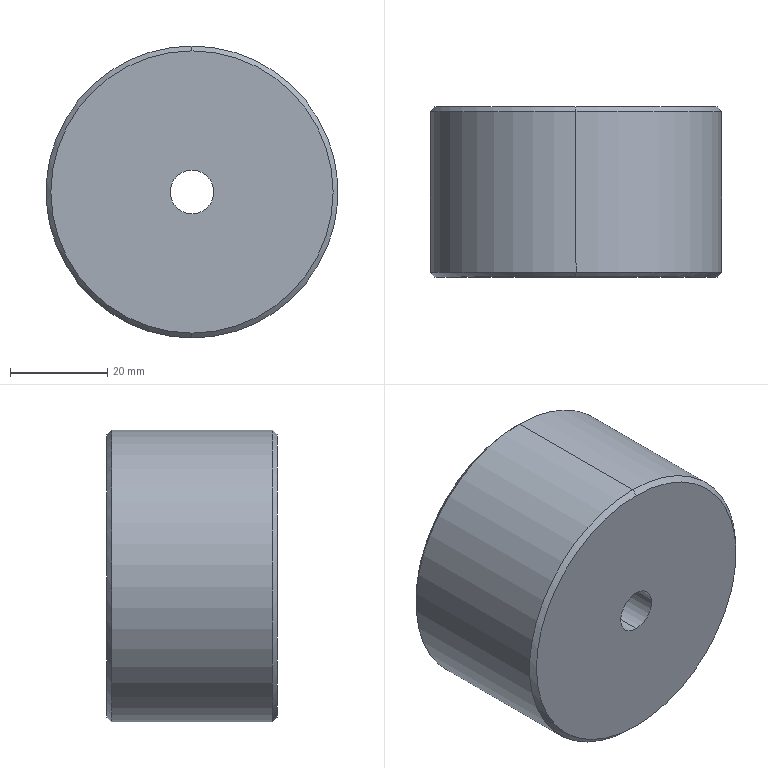Component | SolidWorks | MA060.03.03-10-3 | 1 solid | 15 faces | box 60 x 35 x 60 mm | volume 75578 mm3 | cone 6 | cylinder 6 | plane 3 | commonest cylinder face diameters 15 x2 9 x2 60 x2 | material Polyurethane
build123d program:
from build123d import *

# Parameters (mm, degrees)
SKETCH1_W                                            = 30
SKETCH1_H                                            = 35
HOLE_SIZE_ACCORDING_TO_TYPE_1_OF_HEX_SOC_D           = 9
HOLE_SIZE_ACCORDING_TO_TYPE_1_OF_HEX_SOC_CBORE_D     = 15
HOLE_SIZE_ACCORDING_TO_TYPE_1_OF_HEX_SOC_CBORE_DEPTH = 28
CHAMFER1_SIZE                                        = 20
CHAMFER2_SIZE                                        = 1


with BuildPart() as part:
    # Sketch1 → Revolve1 (revolve)
    with BuildSketch(Plane.XY, mode=Mode.PRIVATE) as revolve1_sk:
        with Locations((15, 17.5)):
            Rectangle(SKETCH1_W, SKETCH1_H)
    revolve(revolve1_sk.sketch.rotate(Axis((0, 0, 0), (0, 1, 0)), 90), axis=Axis((0, 0, 0), (0, 1, 0)))

    # Hole Size According to Type 1 of Hex Soc (through all)
    with Locations(Plane(origin=(0, 35, 0), x_dir=(-1, 0, 0), z_dir=(0, 1, 0))):
        with Locations((0, 0)):
            CounterBoreHole(HOLE_SIZE_ACCORDING_TO_TYPE_1_OF_HEX_SOC_D / 2, HOLE_SIZE_ACCORDING_TO_TYPE_1_OF_HEX_SOC_CBORE_D / 2, HOLE_SIZE_ACCORDING_TO_TYPE_1_OF_HEX_SOC_CBORE_DEPTH)

    # Chamfer1
    chamfer1_edges = [part.edges().sort_by_distance(p)[0] for p in [
        (7.5, 35, 0),
    ]]
    chamfer(chamfer1_edges, length=CHAMFER1_SIZE)

    # Chamfer2
    chamfer2_edges = [part.edges().sort_by_distance(p)[0] for p in [
        (0, 0, 30),
        (0, 35, 30),
    ]]
    chamfer(chamfer2_edges, length=CHAMFER2_SIZE)


solid = part.part

# Placed as in the assembly
solid = solid.moved(Location((263.711, 172.053, -96.036), (0, 0, 0)))
STEP:
#1=COLOUR_RGB('',0.7922,0.8196,0.9333);
#2=FILL_AREA_STYLE_COLOUR('',#1);
#3=FILL_AREA_STYLE('',(#2));
#4=SURFACE_STYLE_FILL_AREA(#3);
#5=SURFACE_SIDE_STYLE('',(#4));
#6=SURFACE_STYLE_USAGE(.BOTH.,#5);
#7=PRESENTATION_STYLE_ASSIGNMENT((#6));
#8=CARTESIAN_POINT('',(10.382,8.152,-4.923));
#9=VERTEX_POINT('',#8);
#10=CARTESIAN_POINT('',(10.382,8.152,-2.639));
#11=VERTEX_POINT('',#10);
#12=CARTESIAN_POINT('',(10.382,8.152,-3.781));
#13=DIRECTION('',(0.,1.,0.));
#14=DIRECTION('',(0.,0.,-1.));
#15=AXIS2_PLACEMENT_3D('',#12,#13,#14);
#16=CIRCLE('',#15,1.142);
#17=EDGE_CURVE('',#9,#11,#16,.T.);
#18=ORIENTED_EDGE('',*,*,#17,.F.);
#19=CARTESIAN_POINT('',(10.382,8.112,-4.962));
#20=VERTEX_POINT('',#19);
#21=CARTESIAN_POINT('',(10.382,8.112,-4.962));
#22=DIRECTION('',(-0.,-0.7071,-0.7071));
#23=VECTOR('',#22,39.37);
#24=LINE('',#21,#23);
#25=EDGE_CURVE('',#9,#20,#24,.T.);
#26=ORIENTED_EDGE('',*,*,#25,.T.);
#27=CARTESIAN_POINT('',(10.382,8.112,-2.6));
#28=VERTEX_POINT('',#27);
#29=CARTESIAN_POINT('',(10.382,8.112,-3.781));
#30=DIRECTION('',(-0.,-1.,-0.));
#31=DIRECTION('',(0.,0.,-1.));
#32=AXIS2_PLACEMENT_3D('',#29,#30,#31);
#33=CIRCLE('',#32,1.181);
#34=EDGE_CURVE('',#28,#20,#33,.T.);
#35=ORIENTED_EDGE('',*,*,#34,.F.);
#36=CARTESIAN_POINT('',(10.382,8.112,-2.6));
#37=DIRECTION('',(-0.,-0.7071,0.7071));
#38=VECTOR('',#37,39.37);
#39=LINE('',#36,#38);
#40=EDGE_CURVE('',#11,#28,#39,.T.);
#41=ORIENTED_EDGE('',*,*,#40,.F.);
#42=EDGE_LOOP('',(#18,#26,#35,#41));
#43=FACE_OUTER_BOUND('',#42,.T.);
#44=CARTESIAN_POINT('',(10.382,8.112,-3.781));
#45=DIRECTION('',(-0.,-1.,-0.));
#46=DIRECTION('',(0.,0.,1.));
#47=AXIS2_PLACEMENT_3D('',#44,#45,#46);
#48=CONICAL_SURFACE('',#47,1.181,0.7854);
#49=ADVANCED_FACE('',(#43),#48,.T.);
#50=CARTESIAN_POINT('',(10.382,6.774,-2.639));
#51=VERTEX_POINT('',#50);
#52=CARTESIAN_POINT('',(10.382,6.774,-4.923));
#53=VERTEX_POINT('',#52);
#54=CARTESIAN_POINT('',(10.382,6.774,-3.781));
#55=DIRECTION('',(-0.,-1.,-0.));
#56=DIRECTION('',(0.,0.,1.));
#57=AXIS2_PLACEMENT_3D('',#54,#55,#56);
#58=CIRCLE('',#57,1.142);
#59=EDGE_CURVE('',#51,#53,#58,.T.);
#60=ORIENTED_EDGE('',*,*,#59,.F.);
#61=CARTESIAN_POINT('',(10.382,6.813,-2.6));
#62=VERTEX_POINT('',#61);
#63=CARTESIAN_POINT('',(10.382,6.774,-2.639));
#64=DIRECTION('',(-0.,0.7071,0.7071));
#65=VECTOR('',#64,39.37);
#66=LINE('',#63,#65);
#67=EDGE_CURVE('',#51,#62,#66,.T.);
#68=ORIENTED_EDGE('',*,*,#67,.T.);
#69=CARTESIAN_POINT('',(10.382,6.813,-4.962));
#70=VERTEX_POINT('',#69);
#71=CARTESIAN_POINT('',(10.382,6.813,-3.781));
#72=DIRECTION('',(0.,1.,0.));
#73=DIRECTION('',(0.,0.,1.));
#74=AXIS2_PLACEMENT_3D('',#71,#72,#73);
#75=CIRCLE('',#74,1.181);
#76=EDGE_CURVE('',#70,#62,#75,.T.);
#77=ORIENTED_EDGE('',*,*,#76,.F.);
#78=CARTESIAN_POINT('',(10.382,6.774,-4.923));
#79=DIRECTION('',(0.,0.7071,-0.7071));
#80=VECTOR('',#79,39.37);
#81=LINE('',#78,#80);
#82=EDGE_CURVE('',#53,#70,#81,.T.);
#83=ORIENTED_EDGE('',*,*,#82,.F.);
#84=EDGE_LOOP('',(#60,#68,#77,#83));
#85=FACE_OUTER_BOUND('',#84,.T.);
#86=CARTESIAN_POINT('',(10.382,6.774,-3.781));
#87=DIRECTION('',(0.,1.,0.));
#88=DIRECTION('',(0.,0.,-1.));
#89=AXIS2_PLACEMENT_3D('',#86,#87,#88);
#90=CONICAL_SURFACE('',#89,1.142,0.7854);
#91=ADVANCED_FACE('',(#85),#90,.T.);
#92=CARTESIAN_POINT('',(10.382,7.364,-3.486));
#93=VERTEX_POINT('',#92);
#94=CARTESIAN_POINT('',(10.382,7.364,-4.076));
#95=VERTEX_POINT('',#94);
#96=CARTESIAN_POINT('',(10.382,7.364,-3.781));
#97=DIRECTION('',(0.,1.,0.));
#98=DIRECTION('',(0.,0.,-1.));
#99=AXIS2_PLACEMENT_3D('',#96,#97,#98);
#100=CIRCLE('',#99,0.2953);
#101=EDGE_CURVE('',#93,#95,#100,.T.);
#102=ORIENTED_EDGE('',*,*,#101,.F.);
#103=CARTESIAN_POINT('',(10.382,8.152,-2.698));
#104=VERTEX_POINT('',#103);
#105=CARTESIAN_POINT('',(10.382,7.364,-3.486));
#106=DIRECTION('',(-0.,0.7071,0.7071));
#107=VECTOR('',#106,39.37);
#108=LINE('',#105,#107);
#109=EDGE_CURVE('',#93,#104,#108,.T.);
#110=ORIENTED_EDGE('',*,*,#109,.T.);
#111=CARTESIAN_POINT('',(10.382,8.152,-4.864));
#112=VERTEX_POINT('',#111);
#113=CARTESIAN_POINT('',(10.382,8.152,-3.781));
#114=DIRECTION('',(-0.,-1.,-0.));
#115=DIRECTION('',(0.,0.,-1.));
#116=AXIS2_PLACEMENT_3D('',#113,#114,#115);
#117=CIRCLE('',#116,1.083);
#118=EDGE_CURVE('',#112,#104,#117,.T.);
#119=ORIENTED_EDGE('',*,*,#118,.F.);
#120=CARTESIAN_POINT('',(10.382,7.364,-4.076));
#121=DIRECTION('',(0.,0.7071,-0.7071));
#122=VECTOR('',#121,39.37);
#123=LINE('',#120,#122);
#124=EDGE_CURVE('',#95,#112,#123,.T.);
#125=ORIENTED_EDGE('',*,*,#124,.F.);
#126=EDGE_LOOP('',(#102,#110,#119,#125));
#127=FACE_OUTER_BOUND('',#126,.T.);
#128=CARTESIAN_POINT('',(10.382,7.364,-3.781));
#129=DIRECTION('',(0.,1.,0.));
#130=DIRECTION('',(0.,0.,-1.));
#131=AXIS2_PLACEMENT_3D('',#128,#129,#130);
#132=CONICAL_SURFACE('',#131,0.2953,0.7854);
#133=ADVANCED_FACE('',(#127),#132,.F.);
#134=CARTESIAN_POINT('',(10.382,7.049,-3.486));
#135=VERTEX_POINT('',#134);
#136=CARTESIAN_POINT('',(10.382,7.049,-4.076));
#137=VERTEX_POINT('',#136);
#138=CARTESIAN_POINT('',(10.382,7.049,-3.781));
#139=DIRECTION('',(0.,1.,0.));
#140=DIRECTION('',(0.,0.,-1.));
#141=AXIS2_PLACEMENT_3D('',#138,#139,#140);
#142=CIRCLE('',#141,0.2953);
#143=EDGE_CURVE('',#135,#137,#142,.T.);
#144=ORIENTED_EDGE('',*,*,#143,.F.);
#145=CARTESIAN_POINT('',(10.382,8.152,-3.486));
#146=DIRECTION('',(0.,1.,0.));
#147=VECTOR('',#146,39.37);
#148=LINE('',#145,#147);
#149=EDGE_CURVE('',#135,#93,#148,.T.);
#150=ORIENTED_EDGE('',*,*,#149,.T.);
#151=ORIENTED_EDGE('',*,*,#101,.T.);
#152=CARTESIAN_POINT('',(10.382,8.152,-4.076));
#153=DIRECTION('',(0.,1.,0.));
#154=VECTOR('',#153,39.37);
#155=LINE('',#152,#154);
#156=EDGE_CURVE('',#137,#95,#155,.T.);
#157=ORIENTED_EDGE('',*,*,#156,.F.);
#158=EDGE_LOOP('',(#144,#150,#151,#157));
#159=FACE_OUTER_BOUND('',#158,.T.);
#160=CARTESIAN_POINT('',(10.382,8.152,-3.781));
#161=DIRECTION('',(0.,1.,0.));
#162=DIRECTION('',(0.,0.,-1.));
#163=AXIS2_PLACEMENT_3D('',#160,#161,#162);
#164=CYLINDRICAL_SURFACE('',#163,0.2953);
#165=ADVANCED_FACE('',(#159),#164,.F.);
#166=CARTESIAN_POINT('',(10.382,6.774,-3.604));
#167=VERTEX_POINT('',#166);
#168=CARTESIAN_POINT('',(10.382,6.774,-3.958));
#169=VERTEX_POINT('',#168);
#170=CARTESIAN_POINT('',(10.382,6.774,-3.781));
#171=DIRECTION('',(0.,1.,0.));
#172=DIRECTION('',(0.,0.,-1.));
#173=AXIS2_PLACEMENT_3D('',#170,#171,#172);
#174=CIRCLE('',#173,0.1772);
#175=EDGE_CURVE('',#167,#169,#174,.T.);
#176=ORIENTED_EDGE('',*,*,#175,.F.);
#177=CARTESIAN_POINT('',(10.382,7.049,-3.604));
#178=VERTEX_POINT('',#177);
#179=CARTESIAN_POINT('',(10.382,8.152,-3.604));
#180=DIRECTION('',(0.,1.,0.));
#181=VECTOR('',#180,39.37);
#182=LINE('',#179,#181);
#183=EDGE_CURVE('',#167,#178,#182,.T.);
#184=ORIENTED_EDGE('',*,*,#183,.T.);
#185=CARTESIAN_POINT('',(10.382,7.049,-3.958));
#186=VERTEX_POINT('',#185);
#187=CARTESIAN_POINT('',(10.382,7.049,-3.781));
#188=DIRECTION('',(0.,1.,0.));
#189=DIRECTION('',(0.,0.,-1.));
#190=AXIS2_PLACEMENT_3D('',#187,#188,#189);
#191=CIRCLE('',#190,0.1772);
#192=EDGE_CURVE('',#178,#186,#191,.T.);
#193=ORIENTED_EDGE('',*,*,#192,.T.);
#194=CARTESIAN_POINT('',(10.382,8.152,-3.958));
#195=DIRECTION('',(0.,1.,0.));
#196=VECTOR('',#195,39.37);
#197=LINE('',#194,#196);
#198=EDGE_CURVE('',#169,#186,#197,.T.);
#199=ORIENTED_EDGE('',*,*,#198,.F.);
#200=EDGE_LOOP('',(#176,#184,#193,#199));
#201=FACE_OUTER_BOUND('',#200,.T.);
#202=CARTESIAN_POINT('',(10.382,8.152,-3.781));
#203=DIRECTION('',(0.,1.,0.));
#204=DIRECTION('',(0.,0.,-1.));
#205=AXIS2_PLACEMENT_3D('',#202,#203,#204);
#206=CYLINDRICAL_SURFACE('',#205,0.1772);
#207=ADVANCED_FACE('',(#201),#206,.F.);
#208=ORIENTED_EDGE('',*,*,#34,.T.);
#209=CARTESIAN_POINT('',(10.382,6.774,-4.962));
#210=DIRECTION('',(-0.,-1.,-0.));
#211=VECTOR('',#210,39.37);
#212=LINE('',#209,#211);
#213=EDGE_CURVE('',#20,#70,#212,.T.);
#214=ORIENTED_EDGE('',*,*,#213,.T.);
#215=ORIENTED_EDGE('',*,*,#76,.T.);
#216=CARTESIAN_POINT('',(10.382,6.774,-2.6));
#217=DIRECTION('',(-0.,-1.,-0.));
#218=VECTOR('',#217,39.37);
#219=LINE('',#216,#218);
#220=EDGE_CURVE('',#28,#62,#219,.T.);
#221=ORIENTED_EDGE('',*,*,#220,.F.);
#222=EDGE_LOOP('',(#208,#214,#215,#221));
#223=FACE_OUTER_BOUND('',#222,.T.);
#224=CARTESIAN_POINT('',(10.382,6.774,-3.781));
#225=DIRECTION('',(-0.,-1.,-0.));
#226=DIRECTION('',(0.,0.,1.));
#227=AXIS2_PLACEMENT_3D('',#224,#225,#226);
#228=CYLINDRICAL_SURFACE('',#227,1.181);
#229=ADVANCED_FACE('',(#223),#228,.T.);
#230=CARTESIAN_POINT('',(10.382,8.152,-3.781));
#231=DIRECTION('',(0.,1.,0.));
#232=DIRECTION('',(0.,0.,-1.));
#233=AXIS2_PLACEMENT_3D('',#230,#231,#232);
#234=CIRCLE('',#233,1.142);
#235=EDGE_CURVE('',#11,#9,#234,.T.);
#236=ORIENTED_EDGE('',*,*,#235,.T.);
#237=ORIENTED_EDGE('',*,*,#17,.T.);
#238=EDGE_LOOP('',(#236,#237));
#239=FACE_OUTER_BOUND('',#238,.T.);
#240=ORIENTED_EDGE('',*,*,#118,.T.);
#241=CARTESIAN_POINT('',(10.382,8.152,-3.781));
#242=DIRECTION('',(-0.,-1.,-0.));
#243=DIRECTION('',(-0.,0.,-1.));
#244=AXIS2_PLACEMENT_3D('',#241,#242,#243);
#245=CIRCLE('',#244,1.083);
#246=EDGE_CURVE('',#104,#112,#245,.T.);
#247=ORIENTED_EDGE('',*,*,#246,.T.);
#248=EDGE_LOOP('',(#240,#247));
#249=FACE_BOUND('',#248,.T.);
#250=CARTESIAN_POINT('',(10.382,8.152,-3.781));
#251=DIRECTION('',(0.,1.,-0.));
#252=DIRECTION('',(0.,-0.,-1.));
#253=AXIS2_PLACEMENT_3D('',#250,#251,#252);
#254=PLANE('',#253);
#255=ADVANCED_FACE('',(#239,#249),#254,.T.);
#256=ORIENTED_EDGE('',*,*,#213,.F.);
#257=CARTESIAN_POINT('',(10.382,8.112,-3.781));
#258=DIRECTION('',(-0.,-1.,-0.));
#259=DIRECTION('',(0.,0.,-1.));
#260=AXIS2_PLACEMENT_3D('',#257,#258,#259);
#261=CIRCLE('',#260,1.181);
#262=EDGE_CURVE('',#20,#28,#261,.T.);
#263=ORIENTED_EDGE('',*,*,#262,.T.);
#264=ORIENTED_EDGE('',*,*,#220,.T.);
#265=CARTESIAN_POINT('',(10.382,6.813,-3.781));
#266=DIRECTION('',(0.,1.,0.));
#267=DIRECTION('',(0.,0.,1.));
#268=AXIS2_PLACEMENT_3D('',#265,#266,#267);
#269=CIRCLE('',#268,1.181);
#270=EDGE_CURVE('',#62,#70,#269,.T.);
#271=ORIENTED_EDGE('',*,*,#270,.T.);
#272=EDGE_LOOP('',(#256,#263,#264,#271));
#273=FACE_OUTER_BOUND('',#272,.T.);
#274=CARTESIAN_POINT('',(10.382,6.774,-3.781));
#275=DIRECTION('',(-0.,-1.,-0.));
#276=DIRECTION('',(0.,0.,1.));
#277=AXIS2_PLACEMENT_3D('',#274,#275,#276);
#278=CYLINDRICAL_SURFACE('',#277,1.181);
#279=ADVANCED_FACE('',(#273),#278,.T.);
#280=CARTESIAN_POINT('',(10.382,6.774,-3.781));
#281=DIRECTION('',(-0.,-1.,-0.));
#282=DIRECTION('',(0.,0.,1.));
#283=AXIS2_PLACEMENT_3D('',#280,#281,#282);
#284=CIRCLE('',#283,1.142);
#285=EDGE_CURVE('',#53,#51,#284,.T.);
#286=ORIENTED_EDGE('',*,*,#285,.T.);
#287=ORIENTED_EDGE('',*,*,#59,.T.);
#288=EDGE_LOOP('',(#286,#287));
#289=FACE_OUTER_BOUND('',#288,.T.);
#290=CARTESIAN_POINT('',(10.382,6.774,-3.781));
#291=DIRECTION('',(0.,1.,0.));
#292=DIRECTION('',(0.,0.,-1.));
#293=AXIS2_PLACEMENT_3D('',#290,#291,#292);
#294=CIRCLE('',#293,0.1772);
#295=EDGE_CURVE('',#169,#167,#294,.T.);
#296=ORIENTED_EDGE('',*,*,#295,.T.);
#297=ORIENTED_EDGE('',*,*,#175,.T.);
#298=EDGE_LOOP('',(#296,#297));
#299=FACE_BOUND('',#298,.T.);
#300=CARTESIAN_POINT('',(10.382,6.774,-3.781));
#301=DIRECTION('',(-0.,-1.,0.));
#302=DIRECTION('',(0.,0.,1.));
#303=AXIS2_PLACEMENT_3D('',#300,#301,#302);
#304=PLANE('',#303);
#305=ADVANCED_FACE('',(#289,#299),#304,.T.);
#306=ORIENTED_EDGE('',*,*,#183,.F.);
#307=ORIENTED_EDGE('',*,*,#295,.F.);
#308=ORIENTED_EDGE('',*,*,#198,.T.);
#309=CARTESIAN_POINT('',(10.382,7.049,-3.781));
#310=DIRECTION('',(0.,1.,0.));
#311=DIRECTION('',(0.,0.,-1.));
#312=AXIS2_PLACEMENT_3D('',#309,#310,#311);
#313=CIRCLE('',#312,0.1772);
#314=EDGE_CURVE('',#186,#178,#313,.T.);
#315=ORIENTED_EDGE('',*,*,#314,.T.);
#316=EDGE_LOOP('',(#306,#307,#308,#315));
#317=FACE_OUTER_BOUND('',#316,.T.);
#318=CARTESIAN_POINT('',(10.382,8.152,-3.781));
#319=DIRECTION('',(0.,1.,0.));
#320=DIRECTION('',(0.,0.,-1.));
#321=AXIS2_PLACEMENT_3D('',#318,#319,#320);
#322=CYLINDRICAL_SURFACE('',#321,0.1772);
#323=ADVANCED_FACE('',(#317),#322,.F.);
#324=ORIENTED_EDGE('',*,*,#314,.F.);
#325=ORIENTED_EDGE('',*,*,#192,.F.);
#326=EDGE_LOOP('',(#324,#325));
#327=FACE_BOUND('',#326,.T.);
#328=CARTESIAN_POINT('',(10.382,7.049,-3.781));
#329=DIRECTION('',(0.,1.,0.));
#330=DIRECTION('',(0.,0.,-1.));
#331=AXIS2_PLACEMENT_3D('',#328,#329,#330);
#332=CIRCLE('',#331,0.2953);
#333=EDGE_CURVE('',#137,#135,#332,.T.);
#334=ORIENTED_EDGE('',*,*,#333,.T.);
#335=ORIENTED_EDGE('',*,*,#143,.T.);
#336=EDGE_LOOP('',(#334,#335));
#337=FACE_OUTER_BOUND('',#336,.T.);
#338=CARTESIAN_POINT('',(10.205,7.049,-3.781));
#339=DIRECTION('',(-0.,-1.,0.));
#340=DIRECTION('',(0.,0.,1.));
#341=AXIS2_PLACEMENT_3D('',#338,#339,#340);
#342=PLANE('',#341);
#343=ADVANCED_FACE('',(#327,#337),#342,.F.);
#344=ORIENTED_EDGE('',*,*,#149,.F.);
#345=ORIENTED_EDGE('',*,*,#333,.F.);
#346=ORIENTED_EDGE('',*,*,#156,.T.);
#347=CARTESIAN_POINT('',(10.382,7.364,-3.781));
#348=DIRECTION('',(0.,1.,0.));
#349=DIRECTION('',(0.,0.,-1.));
#350=AXIS2_PLACEMENT_3D('',#347,#348,#349);
#351=CIRCLE('',#350,0.2953);
#352=EDGE_CURVE('',#95,#93,#351,.T.);
#353=ORIENTED_EDGE('',*,*,#352,.T.);
#354=EDGE_LOOP('',(#344,#345,#346,#353));
#355=FACE_OUTER_BOUND('',#354,.T.);
#356=CARTESIAN_POINT('',(10.382,8.152,-3.781));
#357=DIRECTION('',(0.,1.,0.));
#358=DIRECTION('',(0.,0.,-1.));
#359=AXIS2_PLACEMENT_3D('',#356,#357,#358);
#360=CYLINDRICAL_SURFACE('',#359,0.2953);
#361=ADVANCED_FACE('',(#355),#360,.F.);
#362=ORIENTED_EDGE('',*,*,#109,.F.);
#363=ORIENTED_EDGE('',*,*,#352,.F.);
#364=ORIENTED_EDGE('',*,*,#124,.T.);
#365=ORIENTED_EDGE('',*,*,#246,.F.);
#366=EDGE_LOOP('',(#362,#363,#364,#365));
#367=FACE_OUTER_BOUND('',#366,.T.);
#368=CARTESIAN_POINT('',(10.382,7.364,-3.781));
#369=DIRECTION('',(0.,1.,0.));
#370=DIRECTION('',(0.,0.,-1.));
#371=AXIS2_PLACEMENT_3D('',#368,#369,#370);
#372=CONICAL_SURFACE('',#371,0.2953,0.7854);
#373=ADVANCED_FACE('',(#367),#372,.F.);
#374=ORIENTED_EDGE('',*,*,#67,.F.);
#375=ORIENTED_EDGE('',*,*,#285,.F.);
#376=ORIENTED_EDGE('',*,*,#82,.T.);
#377=ORIENTED_EDGE('',*,*,#270,.F.);
#378=EDGE_LOOP('',(#374,#375,#376,#377));
#379=FACE_OUTER_BOUND('',#378,.T.);
#380=CARTESIAN_POINT('',(10.382,6.774,-3.781));
#381=DIRECTION('',(0.,1.,0.));
#382=DIRECTION('',(0.,0.,-1.));
#383=AXIS2_PLACEMENT_3D('',#380,#381,#382);
#384=CONICAL_SURFACE('',#383,1.142,0.7854);
#385=ADVANCED_FACE('',(#379),#384,.T.);
#386=ORIENTED_EDGE('',*,*,#25,.F.);
#387=ORIENTED_EDGE('',*,*,#235,.F.);
#388=ORIENTED_EDGE('',*,*,#40,.T.);
#389=ORIENTED_EDGE('',*,*,#262,.F.);
#390=EDGE_LOOP('',(#386,#387,#388,#389));
#391=FACE_OUTER_BOUND('',#390,.T.);
#392=CARTESIAN_POINT('',(10.382,8.112,-3.781));
#393=DIRECTION('',(-0.,-1.,-0.));
#394=DIRECTION('',(0.,0.,1.));
#395=AXIS2_PLACEMENT_3D('',#392,#393,#394);
#396=CONICAL_SURFACE('',#395,1.181,0.7854);
#397=ADVANCED_FACE('',(#391),#396,.T.);
#398=CLOSED_SHELL('',(#49,#91,#133,#165,#207,#229,#255,#279,#305,#323,#343,#361,#373,#385,#397));
#399=MANIFOLD_SOLID_BREP('',#398);
#400=STYLED_ITEM('',(#7),#399);
#401=(LENGTH_UNIT()NAMED_UNIT(*)SI_UNIT($,.METRE.));
#402=LENGTH_MEASURE_WITH_UNIT(LENGTH_MEASURE(0.0254),#401);
#403=DIMENSIONAL_EXPONENTS(1.,0.,0.,0.,0.,0.,0.);
#404=(CONVERSION_BASED_UNIT('',#402)LENGTH_UNIT()NAMED_UNIT(#403));
#405=UNCERTAINTY_MEASURE_WITH_UNIT(LENGTH_MEASURE(0.00001),#404,'','');
#406=(NAMED_UNIT(*)PLANE_ANGLE_UNIT()SI_UNIT($,.RADIAN.));
#407=(NAMED_UNIT(*)SI_UNIT($,.STERADIAN.)SOLID_ANGLE_UNIT());
#408=(GEOMETRIC_REPRESENTATION_CONTEXT(3)GLOBAL_UNCERTAINTY_ASSIGNED_CONTEXT((#405))GLOBAL_UNIT_ASSIGNED_CONTEXT((#404,#406,#407))REPRESENTATION_CONTEXT('',''));
#409=MECHANICAL_DESIGN_GEOMETRIC_PRESENTATION_REPRESENTATION('',(#400),#408);
#410=PRESENTATION_LAYER_ASSIGNMENT('','',(#400));
#411=CARTESIAN_POINT('',(0.,0.,0.));
#412=DIRECTION('',(0.,0.,1.));
#413=DIRECTION('',(1.,0.,0.));
#414=AXIS2_PLACEMENT_3D('',#411,#412,#413);
#415=(LENGTH_UNIT()NAMED_UNIT(*)SI_UNIT($,.METRE.));
#416=LENGTH_MEASURE_WITH_UNIT(LENGTH_MEASURE(0.0254),#415);
#417=DIMENSIONAL_EXPONENTS(1.,0.,0.,0.,0.,0.,0.);
#418=(CONVERSION_BASED_UNIT('',#416)LENGTH_UNIT()NAMED_UNIT(#417));
#419=UNCERTAINTY_MEASURE_WITH_UNIT(LENGTH_MEASURE(0.00001),#418,'','');
#420=(NAMED_UNIT(*)PLANE_ANGLE_UNIT()SI_UNIT($,.RADIAN.));
#421=(NAMED_UNIT(*)SI_UNIT($,.STERADIAN.)SOLID_ANGLE_UNIT());
#422=(GEOMETRIC_REPRESENTATION_CONTEXT(3)GLOBAL_UNCERTAINTY_ASSIGNED_CONTEXT((#419))GLOBAL_UNIT_ASSIGNED_CONTEXT((#418,#420,#421))REPRESENTATION_CONTEXT('',''));
#423=ADVANCED_BREP_SHAPE_REPRESENTATION('',(#399,#414),#422);